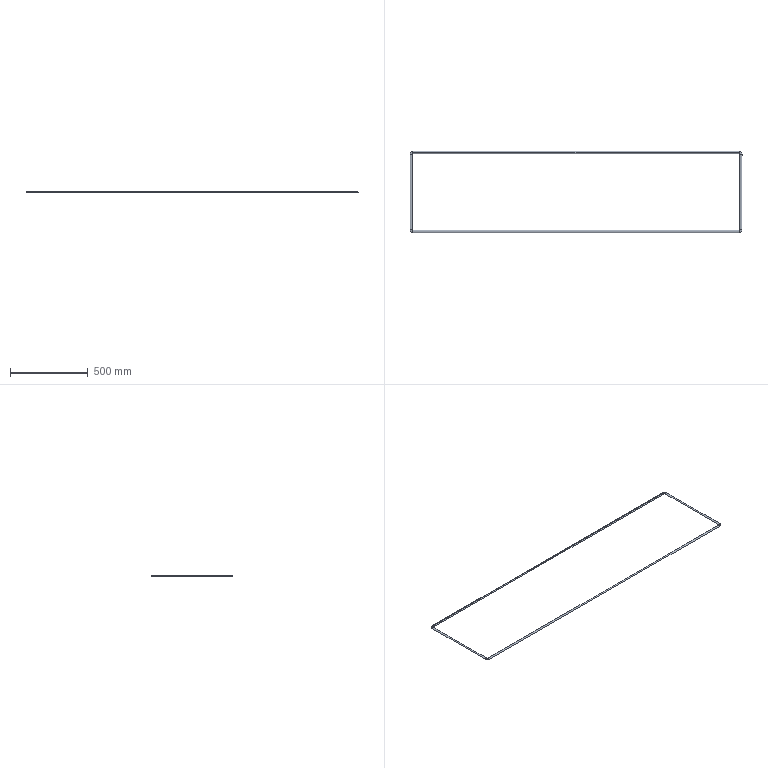Component | SolidWorks | SideDoorAssembly-1_SideDoorSealStrip-1 | 1 solid | 10 faces | volume 106191 mm3 | cylinder 5 | torus 4 | plane 1 | commonest cylinder face diameters 30.125 x5